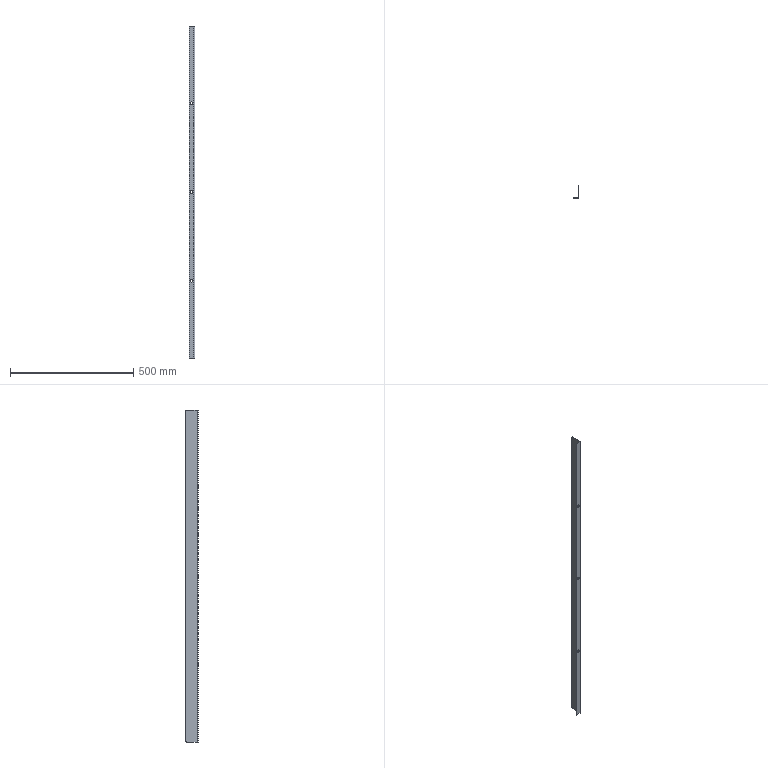Component | SolidWorks | RearRightSidePlateAssembly-1_RearRightSidePlateDoorVerticalRib2-1 | 1 solid | 24 faces | box 24 x 50 x 1345 mm | volume 189730 mm3 | plane 16 | cylinder 8 | commonest cylinder face diameters 10 x6 8 x1 4 x1 | material Plain Carbon Steel
STEP:
#1=COLOUR_RGB('',0.7922,0.8196,0.9333);
#2=FILL_AREA_STYLE_COLOUR('',#1);
#3=FILL_AREA_STYLE('',(#2));
#4=SURFACE_STYLE_FILL_AREA(#3);
#5=SURFACE_SIDE_STYLE('',(#4));
#6=SURFACE_STYLE_USAGE(.BOTH.,#5);
#7=PRESENTATION_STYLE_ASSIGNMENT((#6));
#8=CARTESIAN_POINT('',(96.744,47.699,39.192));
#9=VERTEX_POINT('',#8);
#10=CARTESIAN_POINT('',(96.744,47.699,38.798));
#11=VERTEX_POINT('',#10);
#12=CARTESIAN_POINT('',(96.744,47.699,38.995));
#13=DIRECTION('',(-0.,1.,0.));
#14=DIRECTION('',(0.,0.,-1.));
#15=AXIS2_PLACEMENT_3D('',#12,#13,#14);
#16=CIRCLE('',#15,0.1969);
#17=EDGE_CURVE('',#9,#11,#16,.T.);
#18=ORIENTED_EDGE('',*,*,#17,.F.);
#19=CARTESIAN_POINT('',(96.744,47.778,39.192));
#20=VERTEX_POINT('',#19);
#21=CARTESIAN_POINT('',(96.744,47.699,39.192));
#22=DIRECTION('',(-0.,1.,0.));
#23=VECTOR('',#22,39.37);
#24=LINE('',#21,#23);
#25=EDGE_CURVE('',#9,#20,#24,.T.);
#26=ORIENTED_EDGE('',*,*,#25,.T.);
#27=CARTESIAN_POINT('',(96.744,47.778,38.798));
#28=VERTEX_POINT('',#27);
#29=CARTESIAN_POINT('',(96.744,47.778,38.995));
#30=DIRECTION('',(-0.,1.,0.));
#31=DIRECTION('',(0.,0.,-1.));
#32=AXIS2_PLACEMENT_3D('',#29,#30,#31);
#33=CIRCLE('',#32,0.1969);
#34=EDGE_CURVE('',#20,#28,#33,.T.);
#35=ORIENTED_EDGE('',*,*,#34,.T.);
#36=CARTESIAN_POINT('',(96.744,47.699,38.798));
#37=DIRECTION('',(-0.,1.,0.));
#38=VECTOR('',#37,39.37);
#39=LINE('',#36,#38);
#40=EDGE_CURVE('',#11,#28,#39,.T.);
#41=ORIENTED_EDGE('',*,*,#40,.F.);
#42=EDGE_LOOP('',(#18,#26,#35,#41));
#43=FACE_OUTER_BOUND('',#42,.T.);
#44=CARTESIAN_POINT('',(96.744,47.699,38.995));
#45=DIRECTION('',(-0.,1.,0.));
#46=DIRECTION('',(0.,0.,-1.));
#47=AXIS2_PLACEMENT_3D('',#44,#45,#46);
#48=CYLINDRICAL_SURFACE('',#47,0.1969);
#49=ADVANCED_FACE('',(#43),#48,.F.);
#50=CARTESIAN_POINT('',(96.744,47.699,67.539));
#51=VERTEX_POINT('',#50);
#52=CARTESIAN_POINT('',(96.744,47.699,67.145));
#53=VERTEX_POINT('',#52);
#54=CARTESIAN_POINT('',(96.744,47.699,67.342));
#55=DIRECTION('',(-0.,1.,0.));
#56=DIRECTION('',(0.,0.,-1.));
#57=AXIS2_PLACEMENT_3D('',#54,#55,#56);
#58=CIRCLE('',#57,0.1969);
#59=EDGE_CURVE('',#51,#53,#58,.T.);
#60=ORIENTED_EDGE('',*,*,#59,.F.);
#61=CARTESIAN_POINT('',(96.744,47.778,67.539));
#62=VERTEX_POINT('',#61);
#63=CARTESIAN_POINT('',(96.744,47.699,67.539));
#64=DIRECTION('',(-0.,1.,0.));
#65=VECTOR('',#64,39.37);
#66=LINE('',#63,#65);
#67=EDGE_CURVE('',#51,#62,#66,.T.);
#68=ORIENTED_EDGE('',*,*,#67,.T.);
#69=CARTESIAN_POINT('',(96.744,47.778,67.145));
#70=VERTEX_POINT('',#69);
#71=CARTESIAN_POINT('',(96.744,47.778,67.342));
#72=DIRECTION('',(-0.,1.,0.));
#73=DIRECTION('',(0.,0.,-1.));
#74=AXIS2_PLACEMENT_3D('',#71,#72,#73);
#75=CIRCLE('',#74,0.1969);
#76=EDGE_CURVE('',#62,#70,#75,.T.);
#77=ORIENTED_EDGE('',*,*,#76,.T.);
#78=CARTESIAN_POINT('',(96.744,47.699,67.145));
#79=DIRECTION('',(-0.,1.,0.));
#80=VECTOR('',#79,39.37);
#81=LINE('',#78,#80);
#82=EDGE_CURVE('',#53,#70,#81,.T.);
#83=ORIENTED_EDGE('',*,*,#82,.F.);
#84=EDGE_LOOP('',(#60,#68,#77,#83));
#85=FACE_OUTER_BOUND('',#84,.T.);
#86=CARTESIAN_POINT('',(96.744,47.699,67.342));
#87=DIRECTION('',(-0.,1.,0.));
#88=DIRECTION('',(0.,0.,-1.));
#89=AXIS2_PLACEMENT_3D('',#86,#87,#88);
#90=CYLINDRICAL_SURFACE('',#89,0.1969);
#91=ADVANCED_FACE('',(#85),#90,.F.);
#92=CARTESIAN_POINT('',(96.744,47.699,53.365));
#93=VERTEX_POINT('',#92);
#94=CARTESIAN_POINT('',(96.744,47.699,52.972));
#95=VERTEX_POINT('',#94);
#96=CARTESIAN_POINT('',(96.744,47.699,53.168));
#97=DIRECTION('',(-0.,1.,0.));
#98=DIRECTION('',(0.,0.,-1.));
#99=AXIS2_PLACEMENT_3D('',#96,#97,#98);
#100=CIRCLE('',#99,0.1969);
#101=EDGE_CURVE('',#93,#95,#100,.T.);
#102=ORIENTED_EDGE('',*,*,#101,.F.);
#103=CARTESIAN_POINT('',(96.744,47.778,53.365));
#104=VERTEX_POINT('',#103);
#105=CARTESIAN_POINT('',(96.744,47.699,53.365));
#106=DIRECTION('',(-0.,1.,0.));
#107=VECTOR('',#106,39.37);
#108=LINE('',#105,#107);
#109=EDGE_CURVE('',#93,#104,#108,.T.);
#110=ORIENTED_EDGE('',*,*,#109,.T.);
#111=CARTESIAN_POINT('',(96.744,47.778,52.972));
#112=VERTEX_POINT('',#111);
#113=CARTESIAN_POINT('',(96.744,47.778,53.168));
#114=DIRECTION('',(-0.,1.,0.));
#115=DIRECTION('',(0.,0.,-1.));
#116=AXIS2_PLACEMENT_3D('',#113,#114,#115);
#117=CIRCLE('',#116,0.1969);
#118=EDGE_CURVE('',#104,#112,#117,.T.);
#119=ORIENTED_EDGE('',*,*,#118,.T.);
#120=CARTESIAN_POINT('',(96.744,47.699,52.972));
#121=DIRECTION('',(-0.,1.,0.));
#122=VECTOR('',#121,39.37);
#123=LINE('',#120,#122);
#124=EDGE_CURVE('',#95,#112,#123,.T.);
#125=ORIENTED_EDGE('',*,*,#124,.F.);
#126=EDGE_LOOP('',(#102,#110,#119,#125));
#127=FACE_OUTER_BOUND('',#126,.T.);
#128=CARTESIAN_POINT('',(96.744,47.699,53.168));
#129=DIRECTION('',(-0.,1.,0.));
#130=DIRECTION('',(0.,0.,-1.));
#131=AXIS2_PLACEMENT_3D('',#128,#129,#130);
#132=CYLINDRICAL_SURFACE('',#131,0.1969);
#133=ADVANCED_FACE('',(#127),#132,.F.);
#134=CARTESIAN_POINT('',(97.295,49.581,26.692));
#135=VERTEX_POINT('',#134);
#136=CARTESIAN_POINT('',(97.295,49.581,26.759));
#137=VERTEX_POINT('',#136);
#138=CARTESIAN_POINT('',(97.295,49.581,79.645));
#139=DIRECTION('',(0.,-0.,1.));
#140=VECTOR('',#139,39.37);
#141=LINE('',#138,#140);
#142=EDGE_CURVE('',#135,#137,#141,.T.);
#143=ORIENTED_EDGE('',*,*,#142,.T.);
#144=CARTESIAN_POINT('',(97.295,49.667,26.759));
#145=VERTEX_POINT('',#144);
#146=CARTESIAN_POINT('',(97.295,49.667,26.759));
#147=DIRECTION('',(-0.,1.,0.));
#148=VECTOR('',#147,39.37);
#149=LINE('',#146,#148);
#150=EDGE_CURVE('',#137,#145,#149,.T.);
#151=ORIENTED_EDGE('',*,*,#150,.T.);
#152=CARTESIAN_POINT('',(97.295,49.667,79.578));
#153=VERTEX_POINT('',#152);
#154=CARTESIAN_POINT('',(97.295,49.667,79.645));
#155=DIRECTION('',(-0.,0.,-1.));
#156=VECTOR('',#155,39.37);
#157=LINE('',#154,#156);
#158=EDGE_CURVE('',#153,#145,#157,.T.);
#159=ORIENTED_EDGE('',*,*,#158,.F.);
#160=CARTESIAN_POINT('',(97.295,49.581,79.578));
#161=VERTEX_POINT('',#160);
#162=CARTESIAN_POINT('',(97.295,49.667,79.578));
#163=DIRECTION('',(0.,-1.,-0.));
#164=VECTOR('',#163,39.37);
#165=LINE('',#162,#164);
#166=EDGE_CURVE('',#153,#161,#165,.T.);
#167=ORIENTED_EDGE('',*,*,#166,.T.);
#168=CARTESIAN_POINT('',(97.295,49.581,79.645));
#169=VERTEX_POINT('',#168);
#170=CARTESIAN_POINT('',(97.295,49.581,79.645));
#171=DIRECTION('',(0.,-0.,1.));
#172=VECTOR('',#171,39.37);
#173=LINE('',#170,#172);
#174=EDGE_CURVE('',#161,#169,#173,.T.);
#175=ORIENTED_EDGE('',*,*,#174,.T.);
#176=CARTESIAN_POINT('',(97.295,47.856,79.645));
#177=VERTEX_POINT('',#176);
#178=CARTESIAN_POINT('',(97.295,49.667,79.645));
#179=DIRECTION('',(0.,-1.,-0.));
#180=VECTOR('',#179,39.37);
#181=LINE('',#178,#180);
#182=EDGE_CURVE('',#169,#177,#181,.T.);
#183=ORIENTED_EDGE('',*,*,#182,.T.);
#184=CARTESIAN_POINT('',(97.295,47.856,26.692));
#185=VERTEX_POINT('',#184);
#186=CARTESIAN_POINT('',(97.295,47.856,79.645));
#187=DIRECTION('',(-0.,0.,-1.));
#188=VECTOR('',#187,39.37);
#189=LINE('',#186,#188);
#190=EDGE_CURVE('',#177,#185,#189,.T.);
#191=ORIENTED_EDGE('',*,*,#190,.T.);
#192=CARTESIAN_POINT('',(97.295,49.667,26.692));
#193=DIRECTION('',(0.,-1.,-0.));
#194=VECTOR('',#193,39.37);
#195=LINE('',#192,#194);
#196=EDGE_CURVE('',#135,#185,#195,.T.);
#197=ORIENTED_EDGE('',*,*,#196,.F.);
#198=EDGE_LOOP('',(#143,#151,#159,#167,#175,#183,#191,#197));
#199=FACE_OUTER_BOUND('',#198,.T.);
#200=CARTESIAN_POINT('',(97.295,49.667,79.645));
#201=DIRECTION('',(1.,0.,-0.));
#202=DIRECTION('',(0.,-0.,1.));
#203=AXIS2_PLACEMENT_3D('',#200,#201,#202);
#204=PLANE('',#203);
#205=ADVANCED_FACE('',(#199),#204,.T.);
#206=CARTESIAN_POINT('',(97.137,47.699,79.645));
#207=VERTEX_POINT('',#206);
#208=CARTESIAN_POINT('',(97.137,47.778,79.645));
#209=VERTEX_POINT('',#208);
#210=CARTESIAN_POINT('',(97.137,47.699,79.645));
#211=DIRECTION('',(-0.,1.,0.));
#212=VECTOR('',#211,39.37);
#213=LINE('',#210,#212);
#214=EDGE_CURVE('',#207,#209,#213,.T.);
#215=ORIENTED_EDGE('',*,*,#214,.F.);
#216=CARTESIAN_POINT('',(97.137,47.856,79.645));
#217=DIRECTION('',(-0.,0.,-1.));
#218=DIRECTION('',(-1.,0.,0.));
#219=AXIS2_PLACEMENT_3D('',#216,#217,#218);
#220=CIRCLE('',#219,0.1575);
#221=EDGE_CURVE('',#177,#207,#220,.T.);
#222=ORIENTED_EDGE('',*,*,#221,.F.);
#223=CARTESIAN_POINT('',(97.216,47.856,79.645));
#224=VERTEX_POINT('',#223);
#225=CARTESIAN_POINT('',(97.216,47.856,79.645));
#226=DIRECTION('',(1.,0.,-0.));
#227=VECTOR('',#226,39.37);
#228=LINE('',#225,#227);
#229=EDGE_CURVE('',#224,#177,#228,.T.);
#230=ORIENTED_EDGE('',*,*,#229,.F.);
#231=CARTESIAN_POINT('',(97.137,47.856,79.645));
#232=DIRECTION('',(-0.,0.,-1.));
#233=DIRECTION('',(-1.,0.,0.));
#234=AXIS2_PLACEMENT_3D('',#231,#232,#233);
#235=CIRCLE('',#234,0.07874);
#236=EDGE_CURVE('',#224,#209,#235,.T.);
#237=ORIENTED_EDGE('',*,*,#236,.T.);
#238=EDGE_LOOP('',(#215,#222,#230,#237));
#239=FACE_OUTER_BOUND('',#238,.T.);
#240=CARTESIAN_POINT('',(97.137,47.699,79.645));
#241=DIRECTION('',(0.,-0.,1.));
#242=DIRECTION('',(-1.,-0.,0.));
#243=AXIS2_PLACEMENT_3D('',#240,#241,#242);
#244=PLANE('',#243);
#245=ADVANCED_FACE('',(#239),#244,.T.);
#246=CARTESIAN_POINT('',(96.35,47.699,79.645));
#247=VERTEX_POINT('',#246);
#248=CARTESIAN_POINT('',(97.295,47.699,79.645));
#249=DIRECTION('',(-1.,-0.,0.));
#250=VECTOR('',#249,39.37);
#251=LINE('',#248,#250);
#252=EDGE_CURVE('',#207,#247,#251,.T.);
#253=ORIENTED_EDGE('',*,*,#252,.F.);
#254=ORIENTED_EDGE('',*,*,#214,.T.);
#255=CARTESIAN_POINT('',(96.35,47.778,79.645));
#256=VERTEX_POINT('',#255);
#257=CARTESIAN_POINT('',(97.295,47.778,79.645));
#258=DIRECTION('',(-1.,-0.,0.));
#259=VECTOR('',#258,39.37);
#260=LINE('',#257,#259);
#261=EDGE_CURVE('',#209,#256,#260,.T.);
#262=ORIENTED_EDGE('',*,*,#261,.T.);
#263=CARTESIAN_POINT('',(96.35,47.699,79.645));
#264=DIRECTION('',(-0.,1.,0.));
#265=VECTOR('',#264,39.37);
#266=LINE('',#263,#265);
#267=EDGE_CURVE('',#247,#256,#266,.T.);
#268=ORIENTED_EDGE('',*,*,#267,.F.);
#269=EDGE_LOOP('',(#253,#254,#262,#268));
#270=FACE_OUTER_BOUND('',#269,.T.);
#271=CARTESIAN_POINT('',(97.216,47.856,79.645));
#272=DIRECTION('',(0.,-0.,1.));
#273=DIRECTION('',(-1.,-0.,0.));
#274=AXIS2_PLACEMENT_3D('',#271,#272,#273);
#275=PLANE('',#274);
#276=ADVANCED_FACE('',(#270),#275,.T.);
#277=CARTESIAN_POINT('',(97.216,47.856,26.692));
#278=VERTEX_POINT('',#277);
#279=CARTESIAN_POINT('',(97.295,47.856,26.692));
#280=DIRECTION('',(-1.,-0.,0.));
#281=VECTOR('',#280,39.37);
#282=LINE('',#279,#281);
#283=EDGE_CURVE('',#185,#278,#282,.T.);
#284=ORIENTED_EDGE('',*,*,#283,.F.);
#285=CARTESIAN_POINT('',(97.137,47.699,26.692));
#286=VERTEX_POINT('',#285);
#287=CARTESIAN_POINT('',(97.137,47.856,26.692));
#288=DIRECTION('',(-0.,0.,-1.));
#289=DIRECTION('',(-1.,0.,0.));
#290=AXIS2_PLACEMENT_3D('',#287,#288,#289);
#291=CIRCLE('',#290,0.1575);
#292=EDGE_CURVE('',#185,#286,#291,.T.);
#293=ORIENTED_EDGE('',*,*,#292,.T.);
#294=CARTESIAN_POINT('',(97.137,47.778,26.692));
#295=VERTEX_POINT('',#294);
#296=CARTESIAN_POINT('',(97.137,47.778,26.692));
#297=DIRECTION('',(0.,-1.,-0.));
#298=VECTOR('',#297,39.37);
#299=LINE('',#296,#298);
#300=EDGE_CURVE('',#295,#286,#299,.T.);
#301=ORIENTED_EDGE('',*,*,#300,.F.);
#302=CARTESIAN_POINT('',(97.137,47.856,26.692));
#303=DIRECTION('',(-0.,0.,-1.));
#304=DIRECTION('',(-1.,0.,0.));
#305=AXIS2_PLACEMENT_3D('',#302,#303,#304);
#306=CIRCLE('',#305,0.07874);
#307=EDGE_CURVE('',#278,#295,#306,.T.);
#308=ORIENTED_EDGE('',*,*,#307,.F.);
#309=EDGE_LOOP('',(#284,#293,#301,#308));
#310=FACE_OUTER_BOUND('',#309,.T.);
#311=CARTESIAN_POINT('',(97.295,47.856,26.692));
#312=DIRECTION('',(-0.,0.,-1.));
#313=DIRECTION('',(1.,0.,-0.));
#314=AXIS2_PLACEMENT_3D('',#311,#312,#313);
#315=PLANE('',#314);
#316=ADVANCED_FACE('',(#310),#315,.T.);
#317=CARTESIAN_POINT('',(97.216,49.581,26.692));
#318=VERTEX_POINT('',#317);
#319=CARTESIAN_POINT('',(97.137,49.581,26.692));
#320=DIRECTION('',(-1.,-0.,0.));
#321=VECTOR('',#320,39.37);
#322=LINE('',#319,#321);
#323=EDGE_CURVE('',#135,#318,#322,.T.);
#324=ORIENTED_EDGE('',*,*,#323,.F.);
#325=ORIENTED_EDGE('',*,*,#196,.T.);
#326=ORIENTED_EDGE('',*,*,#283,.T.);
#327=CARTESIAN_POINT('',(97.216,49.667,26.692));
#328=DIRECTION('',(0.,-1.,-0.));
#329=VECTOR('',#328,39.37);
#330=LINE('',#327,#329);
#331=EDGE_CURVE('',#318,#278,#330,.T.);
#332=ORIENTED_EDGE('',*,*,#331,.F.);
#333=EDGE_LOOP('',(#324,#325,#326,#332));
#334=FACE_OUTER_BOUND('',#333,.T.);
#335=CARTESIAN_POINT('',(97.137,47.778,26.692));
#336=DIRECTION('',(-0.,0.,-1.));
#337=DIRECTION('',(1.,0.,-0.));
#338=AXIS2_PLACEMENT_3D('',#335,#336,#337);
#339=PLANE('',#338);
#340=ADVANCED_FACE('',(#334),#339,.T.);
#341=CARTESIAN_POINT('',(96.744,47.778,38.995));
#342=DIRECTION('',(-0.,1.,0.));
#343=DIRECTION('',(0.,0.,-1.));
#344=AXIS2_PLACEMENT_3D('',#341,#342,#343);
#345=CIRCLE('',#344,0.1969);
#346=EDGE_CURVE('',#28,#20,#345,.T.);
#347=ORIENTED_EDGE('',*,*,#346,.F.);
#348=ORIENTED_EDGE('',*,*,#34,.F.);
#349=EDGE_LOOP('',(#347,#348));
#350=FACE_BOUND('',#349,.T.);
#351=CARTESIAN_POINT('',(96.744,47.778,67.342));
#352=DIRECTION('',(-0.,1.,0.));
#353=DIRECTION('',(0.,0.,-1.));
#354=AXIS2_PLACEMENT_3D('',#351,#352,#353);
#355=CIRCLE('',#354,0.1969);
#356=EDGE_CURVE('',#70,#62,#355,.T.);
#357=ORIENTED_EDGE('',*,*,#356,.F.);
#358=ORIENTED_EDGE('',*,*,#76,.F.);
#359=EDGE_LOOP('',(#357,#358));
#360=FACE_BOUND('',#359,.T.);
#361=CARTESIAN_POINT('',(96.744,47.778,53.168));
#362=DIRECTION('',(-0.,1.,0.));
#363=DIRECTION('',(0.,0.,-1.));
#364=AXIS2_PLACEMENT_3D('',#361,#362,#363);
#365=CIRCLE('',#364,0.1969);
#366=EDGE_CURVE('',#112,#104,#365,.T.);
#367=ORIENTED_EDGE('',*,*,#366,.F.);
#368=ORIENTED_EDGE('',*,*,#118,.F.);
#369=EDGE_LOOP('',(#367,#368));
#370=FACE_BOUND('',#369,.T.);
#371=CARTESIAN_POINT('',(96.35,47.778,26.692));
#372=VERTEX_POINT('',#371);
#373=CARTESIAN_POINT('',(97.295,47.778,26.692));
#374=DIRECTION('',(-1.,-0.,0.));
#375=VECTOR('',#374,39.37);
#376=LINE('',#373,#375);
#377=EDGE_CURVE('',#295,#372,#376,.T.);
#378=ORIENTED_EDGE('',*,*,#377,.T.);
#379=CARTESIAN_POINT('',(96.35,47.778,79.645));
#380=DIRECTION('',(-0.,0.,-1.));
#381=VECTOR('',#380,39.37);
#382=LINE('',#379,#381);
#383=EDGE_CURVE('',#256,#372,#382,.T.);
#384=ORIENTED_EDGE('',*,*,#383,.F.);
#385=ORIENTED_EDGE('',*,*,#261,.F.);
#386=CARTESIAN_POINT('',(97.137,47.778,79.645));
#387=DIRECTION('',(-0.,0.,-1.));
#388=VECTOR('',#387,39.37);
#389=LINE('',#386,#388);
#390=EDGE_CURVE('',#209,#295,#389,.T.);
#391=ORIENTED_EDGE('',*,*,#390,.T.);
#392=EDGE_LOOP('',(#378,#384,#385,#391));
#393=FACE_OUTER_BOUND('',#392,.T.);
#394=CARTESIAN_POINT('',(97.295,47.778,79.645));
#395=DIRECTION('',(0.,-1.,-0.));
#396=DIRECTION('',(0.,-0.,1.));
#397=AXIS2_PLACEMENT_3D('',#394,#395,#396);
#398=PLANE('',#397);
#399=ADVANCED_FACE('',(#350,#360,#370,#393),#398,.F.);
#400=CARTESIAN_POINT('',(96.35,47.699,26.692));
#401=VERTEX_POINT('',#400);
#402=CARTESIAN_POINT('',(96.35,47.699,26.692));
#403=DIRECTION('',(-0.,1.,0.));
#404=VECTOR('',#403,39.37);
#405=LINE('',#402,#404);
#406=EDGE_CURVE('',#401,#372,#405,.T.);
#407=ORIENTED_EDGE('',*,*,#406,.F.);
#408=CARTESIAN_POINT('',(96.35,47.699,79.645));
#409=DIRECTION('',(-0.,0.,-1.));
#410=VECTOR('',#409,39.37);
#411=LINE('',#408,#410);
#412=EDGE_CURVE('',#247,#401,#411,.T.);
#413=ORIENTED_EDGE('',*,*,#412,.F.);
#414=ORIENTED_EDGE('',*,*,#267,.T.);
#415=ORIENTED_EDGE('',*,*,#383,.T.);
#416=EDGE_LOOP('',(#407,#413,#414,#415));
#417=FACE_OUTER_BOUND('',#416,.T.);
#418=CARTESIAN_POINT('',(96.35,47.699,79.645));
#419=DIRECTION('',(-1.,-0.,0.));
#420=DIRECTION('',(-0.,0.,-1.));
#421=AXIS2_PLACEMENT_3D('',#418,#419,#420);
#422=PLANE('',#421);
#423=ADVANCED_FACE('',(#417),#422,.T.);
#424=CARTESIAN_POINT('',(96.744,47.699,38.995));
#425=DIRECTION('',(-0.,1.,0.));
#426=DIRECTION('',(0.,0.,-1.));
#427=AXIS2_PLACEMENT_3D('',#424,#425,#426);
#428=CIRCLE('',#427,0.1969);
#429=EDGE_CURVE('',#11,#9,#428,.T.);
#430=ORIENTED_EDGE('',*,*,#429,.T.);
#431=ORIENTED_EDGE('',*,*,#17,.T.);
#432=EDGE_LOOP('',(#430,#431));
#433=FACE_BOUND('',#432,.T.);
#434=CARTESIAN_POINT('',(96.744,47.699,67.342));
#435=DIRECTION('',(-0.,1.,0.));
#436=DIRECTION('',(0.,0.,-1.));
#437=AXIS2_PLACEMENT_3D('',#434,#435,#436);
#438=CIRCLE('',#437,0.1969);
#439=EDGE_CURVE('',#53,#51,#438,.T.);
#440=ORIENTED_EDGE('',*,*,#439,.T.);
#441=ORIENTED_EDGE('',*,*,#59,.T.);
#442=EDGE_LOOP('',(#440,#441));
#443=FACE_BOUND('',#442,.T.);
#444=CARTESIAN_POINT('',(96.744,47.699,53.168));
#445=DIRECTION('',(-0.,1.,0.));
#446=DIRECTION('',(0.,0.,-1.));
#447=AXIS2_PLACEMENT_3D('',#444,#445,#446);
#448=CIRCLE('',#447,0.1969);
#449=EDGE_CURVE('',#95,#93,#448,.T.);
#450=ORIENTED_EDGE('',*,*,#449,.T.);
#451=ORIENTED_EDGE('',*,*,#101,.T.);
#452=EDGE_LOOP('',(#450,#451));
#453=FACE_BOUND('',#452,.T.);
#454=CARTESIAN_POINT('',(97.295,47.699,26.692));
#455=DIRECTION('',(-1.,-0.,0.));
#456=VECTOR('',#455,39.37);
#457=LINE('',#454,#456);
#458=EDGE_CURVE('',#286,#401,#457,.T.);
#459=ORIENTED_EDGE('',*,*,#458,.F.);
#460=CARTESIAN_POINT('',(97.137,47.699,79.645));
#461=DIRECTION('',(-0.,0.,-1.));
#462=VECTOR('',#461,39.37);
#463=LINE('',#460,#462);
#464=EDGE_CURVE('',#207,#286,#463,.T.);
#465=ORIENTED_EDGE('',*,*,#464,.F.);
#466=ORIENTED_EDGE('',*,*,#252,.T.);
#467=ORIENTED_EDGE('',*,*,#412,.T.);
#468=EDGE_LOOP('',(#459,#465,#466,#467));
#469=FACE_OUTER_BOUND('',#468,.T.);
#470=CARTESIAN_POINT('',(97.295,47.699,79.645));
#471=DIRECTION('',(0.,-1.,-0.));
#472=DIRECTION('',(0.,-0.,1.));
#473=AXIS2_PLACEMENT_3D('',#470,#471,#472);
#474=PLANE('',#473);
#475=ADVANCED_FACE('',(#433,#443,#453,#469),#474,.T.);
#476=ORIENTED_EDGE('',*,*,#292,.F.);
#477=ORIENTED_EDGE('',*,*,#190,.F.);
#478=ORIENTED_EDGE('',*,*,#221,.T.);
#479=ORIENTED_EDGE('',*,*,#464,.T.);
#480=EDGE_LOOP('',(#476,#477,#478,#479));
#481=FACE_OUTER_BOUND('',#480,.T.);
#482=CARTESIAN_POINT('',(97.137,47.856,79.645));
#483=DIRECTION('',(-0.,0.,-1.));
#484=DIRECTION('',(1.,0.,0.));
#485=AXIS2_PLACEMENT_3D('',#482,#483,#484);
#486=CYLINDRICAL_SURFACE('',#485,0.1575);
#487=ADVANCED_FACE('',(#481),#486,.T.);
#488=CARTESIAN_POINT('',(97.216,49.667,26.759));
#489=VERTEX_POINT('',#488);
#490=CARTESIAN_POINT('',(97.216,49.667,26.759));
#491=DIRECTION('',(1.,0.,-0.));
#492=VECTOR('',#491,39.37);
#493=LINE('',#490,#492);
#494=EDGE_CURVE('',#489,#145,#493,.T.);
#495=ORIENTED_EDGE('',*,*,#494,.F.);
#496=CARTESIAN_POINT('',(97.216,49.667,79.578));
#497=VERTEX_POINT('',#496);
#498=CARTESIAN_POINT('',(97.216,49.667,79.645));
#499=DIRECTION('',(-0.,0.,-1.));
#500=VECTOR('',#499,39.37);
#501=LINE('',#498,#500);
#502=EDGE_CURVE('',#497,#489,#501,.T.);
#503=ORIENTED_EDGE('',*,*,#502,.F.);
#504=CARTESIAN_POINT('',(97.216,49.667,79.578));
#505=DIRECTION('',(-1.,-0.,0.));
#506=VECTOR('',#505,39.37);
#507=LINE('',#504,#506);
#508=EDGE_CURVE('',#153,#497,#507,.T.);
#509=ORIENTED_EDGE('',*,*,#508,.F.);
#510=ORIENTED_EDGE('',*,*,#158,.T.);
#511=EDGE_LOOP('',(#495,#503,#509,#510));
#512=FACE_OUTER_BOUND('',#511,.T.);
#513=CARTESIAN_POINT('',(97.216,49.667,79.645));
#514=DIRECTION('',(-0.,1.,0.));
#515=DIRECTION('',(-0.,0.,-1.));
#516=AXIS2_PLACEMENT_3D('',#513,#514,#515);
#517=PLANE('',#516);
#518=ADVANCED_FACE('',(#512),#517,.T.);
#519=ORIENTED_EDGE('',*,*,#502,.T.);
#520=CARTESIAN_POINT('',(97.216,49.581,26.759));
#521=VERTEX_POINT('',#520);
#522=CARTESIAN_POINT('',(97.216,49.667,26.759));
#523=DIRECTION('',(0.,-1.,-0.));
#524=VECTOR('',#523,39.37);
#525=LINE('',#522,#524);
#526=EDGE_CURVE('',#489,#521,#525,.T.);
#527=ORIENTED_EDGE('',*,*,#526,.T.);
#528=CARTESIAN_POINT('',(97.216,49.581,79.645));
#529=DIRECTION('',(-0.,0.,-1.));
#530=VECTOR('',#529,39.37);
#531=LINE('',#528,#530);
#532=EDGE_CURVE('',#521,#318,#531,.T.);
#533=ORIENTED_EDGE('',*,*,#532,.T.);
#534=ORIENTED_EDGE('',*,*,#331,.T.);
#535=CARTESIAN_POINT('',(97.216,47.856,79.645));
#536=DIRECTION('',(-0.,0.,-1.));
#537=VECTOR('',#536,39.37);
#538=LINE('',#535,#537);
#539=EDGE_CURVE('',#224,#278,#538,.T.);
#540=ORIENTED_EDGE('',*,*,#539,.F.);
#541=CARTESIAN_POINT('',(97.216,49.581,79.645));
#542=VERTEX_POINT('',#541);
#543=CARTESIAN_POINT('',(97.216,49.667,79.645));
#544=DIRECTION('',(0.,-1.,-0.));
#545=VECTOR('',#544,39.37);
#546=LINE('',#543,#545);
#547=EDGE_CURVE('',#542,#224,#546,.T.);
#548=ORIENTED_EDGE('',*,*,#547,.F.);
#549=CARTESIAN_POINT('',(97.216,49.581,79.578));
#550=VERTEX_POINT('',#549);
#551=CARTESIAN_POINT('',(97.216,49.581,79.645));
#552=DIRECTION('',(-0.,0.,-1.));
#553=VECTOR('',#552,39.37);
#554=LINE('',#551,#553);
#555=EDGE_CURVE('',#542,#550,#554,.T.);
#556=ORIENTED_EDGE('',*,*,#555,.T.);
#557=CARTESIAN_POINT('',(97.216,49.667,79.578));
#558=DIRECTION('',(-0.,1.,0.));
#559=VECTOR('',#558,39.37);
#560=LINE('',#557,#559);
#561=EDGE_CURVE('',#550,#497,#560,.T.);
#562=ORIENTED_EDGE('',*,*,#561,.T.);
#563=EDGE_LOOP('',(#519,#527,#533,#534,#540,#548,#556,#562));
#564=FACE_OUTER_BOUND('',#563,.T.);
#565=CARTESIAN_POINT('',(97.216,49.667,79.645));
#566=DIRECTION('',(1.,0.,-0.));
#567=DIRECTION('',(0.,-0.,1.));
#568=AXIS2_PLACEMENT_3D('',#565,#566,#567);
#569=PLANE('',#568);
#570=ADVANCED_FACE('',(#564),#569,.F.);
#571=ORIENTED_EDGE('',*,*,#307,.T.);
#572=ORIENTED_EDGE('',*,*,#390,.F.);
#573=ORIENTED_EDGE('',*,*,#236,.F.);
#574=ORIENTED_EDGE('',*,*,#539,.T.);
#575=EDGE_LOOP('',(#571,#572,#573,#574));
#576=FACE_OUTER_BOUND('',#575,.T.);
#577=CARTESIAN_POINT('',(97.137,47.856,79.645));
#578=DIRECTION('',(-0.,0.,-1.));
#579=DIRECTION('',(1.,0.,0.));
#580=AXIS2_PLACEMENT_3D('',#577,#578,#579);
#581=CYLINDRICAL_SURFACE('',#580,0.07874);
#582=ADVANCED_FACE('',(#576),#581,.F.);
#583=CARTESIAN_POINT('',(97.137,49.581,79.645));
#584=DIRECTION('',(1.,0.,-0.));
#585=VECTOR('',#584,39.37);
#586=LINE('',#583,#585);
#587=EDGE_CURVE('',#542,#169,#586,.T.);
#588=ORIENTED_EDGE('',*,*,#587,.F.);
#589=ORIENTED_EDGE('',*,*,#547,.T.);
#590=ORIENTED_EDGE('',*,*,#229,.T.);
#591=ORIENTED_EDGE('',*,*,#182,.F.);
#592=EDGE_LOOP('',(#588,#589,#590,#591));
#593=FACE_OUTER_BOUND('',#592,.T.);
#594=CARTESIAN_POINT('',(97.137,47.856,79.645));
#595=DIRECTION('',(0.,-0.,1.));
#596=DIRECTION('',(-1.,-0.,0.));
#597=AXIS2_PLACEMENT_3D('',#594,#595,#596);
#598=PLANE('',#597);
#599=ADVANCED_FACE('',(#593),#598,.T.);
#600=ORIENTED_EDGE('',*,*,#377,.F.);
#601=ORIENTED_EDGE('',*,*,#300,.T.);
#602=ORIENTED_EDGE('',*,*,#458,.T.);
#603=ORIENTED_EDGE('',*,*,#406,.T.);
#604=EDGE_LOOP('',(#600,#601,#602,#603));
#605=FACE_OUTER_BOUND('',#604,.T.);
#606=CARTESIAN_POINT('',(97.137,47.856,26.692));
#607=DIRECTION('',(0.,-0.,1.));
#608=DIRECTION('',(-1.,-0.,0.));
#609=AXIS2_PLACEMENT_3D('',#606,#607,#608);
#610=PLANE('',#609);
#611=ADVANCED_FACE('',(#605),#610,.F.);
#612=ORIENTED_EDGE('',*,*,#109,.F.);
#613=ORIENTED_EDGE('',*,*,#449,.F.);
#614=ORIENTED_EDGE('',*,*,#124,.T.);
#615=ORIENTED_EDGE('',*,*,#366,.T.);
#616=EDGE_LOOP('',(#612,#613,#614,#615));
#617=FACE_OUTER_BOUND('',#616,.T.);
#618=CARTESIAN_POINT('',(96.744,47.699,53.168));
#619=DIRECTION('',(-0.,1.,0.));
#620=DIRECTION('',(0.,0.,-1.));
#621=AXIS2_PLACEMENT_3D('',#618,#619,#620);
#622=CYLINDRICAL_SURFACE('',#621,0.1969);
#623=ADVANCED_FACE('',(#617),#622,.F.);
#624=ORIENTED_EDGE('',*,*,#67,.F.);
#625=ORIENTED_EDGE('',*,*,#439,.F.);
#626=ORIENTED_EDGE('',*,*,#82,.T.);
#627=ORIENTED_EDGE('',*,*,#356,.T.);
#628=EDGE_LOOP('',(#624,#625,#626,#627));
#629=FACE_OUTER_BOUND('',#628,.T.);
#630=CARTESIAN_POINT('',(96.744,47.699,67.342));
#631=DIRECTION('',(-0.,1.,0.));
#632=DIRECTION('',(0.,0.,-1.));
#633=AXIS2_PLACEMENT_3D('',#630,#631,#632);
#634=CYLINDRICAL_SURFACE('',#633,0.1969);
#635=ADVANCED_FACE('',(#629),#634,.F.);
#636=ORIENTED_EDGE('',*,*,#25,.F.);
#637=ORIENTED_EDGE('',*,*,#429,.F.);
#638=ORIENTED_EDGE('',*,*,#40,.T.);
#639=ORIENTED_EDGE('',*,*,#346,.T.);
#640=EDGE_LOOP('',(#636,#637,#638,#639));
#641=FACE_OUTER_BOUND('',#640,.T.);
#642=CARTESIAN_POINT('',(96.744,47.699,38.995));
#643=DIRECTION('',(-0.,1.,0.));
#644=DIRECTION('',(0.,0.,-1.));
#645=AXIS2_PLACEMENT_3D('',#642,#643,#644);
#646=CYLINDRICAL_SURFACE('',#645,0.1969);
#647=ADVANCED_FACE('',(#641),#646,.F.);
#648=ORIENTED_EDGE('',*,*,#587,.T.);
#649=ORIENTED_EDGE('',*,*,#174,.F.);
#650=CARTESIAN_POINT('',(97.295,49.581,79.578));
#651=DIRECTION('',(-1.,-0.,0.));
#652=VECTOR('',#651,39.37);
#653=LINE('',#650,#652);
#654=EDGE_CURVE('',#161,#550,#653,.T.);
#655=ORIENTED_EDGE('',*,*,#654,.T.);
#656=ORIENTED_EDGE('',*,*,#555,.F.);
#657=EDGE_LOOP('',(#648,#649,#655,#656));
#658=FACE_OUTER_BOUND('',#657,.T.);
#659=CARTESIAN_POINT('',(97.295,49.581,79.578));
#660=DIRECTION('',(0.,-1.,-0.));
#661=DIRECTION('',(0.,-0.,1.));
#662=AXIS2_PLACEMENT_3D('',#659,#660,#661);
#663=PLANE('',#662);
#664=ADVANCED_FACE('',(#658),#663,.F.);
#665=ORIENTED_EDGE('',*,*,#508,.T.);
#666=ORIENTED_EDGE('',*,*,#561,.F.);
#667=ORIENTED_EDGE('',*,*,#654,.F.);
#668=ORIENTED_EDGE('',*,*,#166,.F.);
#669=EDGE_LOOP('',(#665,#666,#667,#668));
#670=FACE_OUTER_BOUND('',#669,.T.);
#671=CARTESIAN_POINT('',(97.295,49.693,79.578));
#672=DIRECTION('',(-0.,0.,-1.));
#673=DIRECTION('',(1.,0.,-0.));
#674=AXIS2_PLACEMENT_3D('',#671,#672,#673);
#675=PLANE('',#674);
#676=ADVANCED_FACE('',(#670),#675,.F.);
#677=ORIENTED_EDGE('',*,*,#494,.T.);
#678=ORIENTED_EDGE('',*,*,#150,.F.);
#679=CARTESIAN_POINT('',(97.295,49.581,26.759));
#680=DIRECTION('',(-1.,-0.,0.));
#681=VECTOR('',#680,39.37);
#682=LINE('',#679,#681);
#683=EDGE_CURVE('',#137,#521,#682,.T.);
#684=ORIENTED_EDGE('',*,*,#683,.T.);
#685=ORIENTED_EDGE('',*,*,#526,.F.);
#686=EDGE_LOOP('',(#677,#678,#684,#685));
#687=FACE_OUTER_BOUND('',#686,.T.);
#688=CARTESIAN_POINT('',(97.295,49.693,26.759));
#689=DIRECTION('',(0.,-0.,1.));
#690=DIRECTION('',(-1.,-0.,0.));
#691=AXIS2_PLACEMENT_3D('',#688,#689,#690);
#692=PLANE('',#691);
#693=ADVANCED_FACE('',(#687),#692,.F.);
#694=ORIENTED_EDGE('',*,*,#323,.T.);
#695=ORIENTED_EDGE('',*,*,#532,.F.);
#696=ORIENTED_EDGE('',*,*,#683,.F.);
#697=ORIENTED_EDGE('',*,*,#142,.F.);
#698=EDGE_LOOP('',(#694,#695,#696,#697));
#699=FACE_OUTER_BOUND('',#698,.T.);
#700=CARTESIAN_POINT('',(97.295,49.581,26.673));
#701=DIRECTION('',(0.,-1.,-0.));
#702=DIRECTION('',(0.,-0.,1.));
#703=AXIS2_PLACEMENT_3D('',#700,#701,#702);
#704=PLANE('',#703);
#705=ADVANCED_FACE('',(#699),#704,.F.);
#706=CLOSED_SHELL('',(#49,#91,#133,#205,#245,#276,#316,#340,#399,#423,#475,#487,#518,#570,#582,#599,#611,#623,#635,#647,#664,#676,#693,#705));
#707=MANIFOLD_SOLID_BREP('',#706);
#708=STYLED_ITEM('',(#7),#707);
#709=(LENGTH_UNIT()NAMED_UNIT(*)SI_UNIT($,.METRE.));
#710=LENGTH_MEASURE_WITH_UNIT(LENGTH_MEASURE(0.0254),#709);
#711=DIMENSIONAL_EXPONENTS(1.,0.,0.,0.,0.,0.,0.);
#712=(CONVERSION_BASED_UNIT('',#710)LENGTH_UNIT()NAMED_UNIT(#711));
#713=UNCERTAINTY_MEASURE_WITH_UNIT(LENGTH_MEASURE(0.00001),#712,'','');
#714=(NAMED_UNIT(*)PLANE_ANGLE_UNIT()SI_UNIT($,.RADIAN.));
#715=(NAMED_UNIT(*)SI_UNIT($,.STERADIAN.)SOLID_ANGLE_UNIT());
#716=(GEOMETRIC_REPRESENTATION_CONTEXT(3)GLOBAL_UNCERTAINTY_ASSIGNED_CONTEXT((#713))GLOBAL_UNIT_ASSIGNED_CONTEXT((#712,#714,#715))REPRESENTATION_CONTEXT('',''));
#717=MECHANICAL_DESIGN_GEOMETRIC_PRESENTATION_REPRESENTATION('',(#708),#716);
#718=CARTESIAN_POINT('',(0.,0.,0.));
#719=DIRECTION('',(0.,0.,1.));
#720=DIRECTION('',(1.,0.,0.));
#721=AXIS2_PLACEMENT_3D('',#718,#719,#720);
#722=(LENGTH_UNIT()NAMED_UNIT(*)SI_UNIT($,.METRE.));
#723=LENGTH_MEASURE_WITH_UNIT(LENGTH_MEASURE(0.0254),#722);
#724=DIMENSIONAL_EXPONENTS(1.,0.,0.,0.,0.,0.,0.);
#725=(CONVERSION_BASED_UNIT('',#723)LENGTH_UNIT()NAMED_UNIT(#724));
#726=UNCERTAINTY_MEASURE_WITH_UNIT(LENGTH_MEASURE(0.00001),#725,'','');
#727=(NAMED_UNIT(*)PLANE_ANGLE_UNIT()SI_UNIT($,.RADIAN.));
#728=(NAMED_UNIT(*)SI_UNIT($,.STERADIAN.)SOLID_ANGLE_UNIT());
#729=(GEOMETRIC_REPRESENTATION_CONTEXT(3)GLOBAL_UNCERTAINTY_ASSIGNED_CONTEXT((#726))GLOBAL_UNIT_ASSIGNED_CONTEXT((#725,#727,#728))REPRESENTATION_CONTEXT('',''));
#730=ADVANCED_BREP_SHAPE_REPRESENTATION('',(#707,#721),#729);
#731=PRESENTATION_LAYER_ASSIGNMENT('','',(#708));